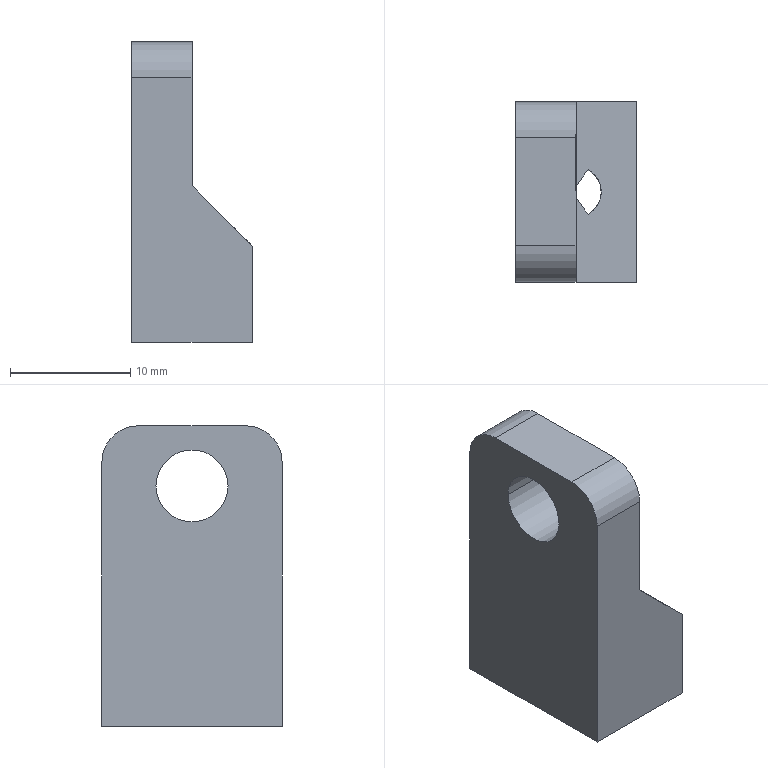Component | SolidWorks | UpperHinge-1 | 1 solid | 15 faces | box 10 x 15 x 25 mm | volume 2332 mm3 | plane 8 | cylinder 6 | cone 1 | commonest cylinder face diameters 6 x4 4.2 x2
STEP:
#1=COLOUR_RGB('',0.7922,0.8196,0.9333);
#2=FILL_AREA_STYLE_COLOUR('',#1);
#3=FILL_AREA_STYLE('',(#2));
#4=SURFACE_STYLE_FILL_AREA(#3);
#5=SURFACE_SIDE_STYLE('',(#4));
#6=SURFACE_STYLE_USAGE(.BOTH.,#5);
#7=PRESENTATION_STYLE_ASSIGNMENT((#6));
#8=CARTESIAN_POINT('',(-0.1614,-8.631,3.169));
#9=VERTEX_POINT('',#8);
#10=CARTESIAN_POINT('',(-0.03937,-8.558,3.169));
#11=VERTEX_POINT('',#10);
#12=CARTESIAN_POINT('',(-0.07874,-8.631,3.169));
#13=DIRECTION('',(0.,0.,-1.));
#14=DIRECTION('',(1.,0.,0.));
#15=AXIS2_PLACEMENT_3D('',#12,#13,#14);
#16=CIRCLE('',#15,0.08268);
#17=EDGE_CURVE('',#9,#11,#16,.T.);
#18=ORIENTED_EDGE('',*,*,#17,.F.);
#19=CARTESIAN_POINT('',(-0.1614,-8.631,2.697));
#20=VERTEX_POINT('',#19);
#21=CARTESIAN_POINT('',(-0.1614,-8.631,2.697));
#22=DIRECTION('',(0.,0.,-1.));
#23=VECTOR('',#22,39.37);
#24=LINE('',#21,#23);
#25=EDGE_CURVE('',#9,#20,#24,.T.);
#26=ORIENTED_EDGE('',*,*,#25,.T.);
#27=CARTESIAN_POINT('',(0.003937,-8.631,2.697));
#28=VERTEX_POINT('',#27);
#29=CARTESIAN_POINT('',(-0.07874,-8.631,2.697));
#30=DIRECTION('',(0.,0.,-1.));
#31=DIRECTION('',(1.,0.,0.));
#32=AXIS2_PLACEMENT_3D('',#29,#30,#31);
#33=CIRCLE('',#32,0.08268);
#34=EDGE_CURVE('',#20,#28,#33,.T.);
#35=ORIENTED_EDGE('',*,*,#34,.T.);
#36=CARTESIAN_POINT('',(0.003937,-8.631,3.126));
#37=VERTEX_POINT('',#36);
#38=CARTESIAN_POINT('',(0.003937,-8.631,2.697));
#39=DIRECTION('',(0.,0.,-1.));
#40=VECTOR('',#39,39.37);
#41=LINE('',#38,#40);
#42=EDGE_CURVE('',#37,#28,#41,.T.);
#43=ORIENTED_EDGE('',*,*,#42,.F.);
#44=CARTESIAN_POINT('',(0.003937,-8.631,3.126));
#45=CARTESIAN_POINT('',(0.003937,-8.6,3.126));
#46=CARTESIAN_POINT('',(-0.01199,-8.573,3.142));
#47=CARTESIAN_POINT('',(-0.03937,-8.558,3.169));
#48=(BOUNDED_CURVE()B_SPLINE_CURVE(3,(#44,#45,#46,#47),.UNSPECIFIED.,.F.,.F.)B_SPLINE_CURVE_WITH_KNOTS((4,4),(0.,1.074),.UNSPECIFIED.)CURVE()GEOMETRIC_REPRESENTATION_ITEM()RATIONAL_B_SPLINE_CURVE((1.,0.9061,0.9061,1.))REPRESENTATION_ITEM(''));
#49=EDGE_CURVE('',#37,#11,#48,.T.);
#50=ORIENTED_EDGE('',*,*,#49,.T.);
#51=EDGE_LOOP('',(#18,#26,#35,#43,#50));
#52=FACE_OUTER_BOUND('',#51,.T.);
#53=CARTESIAN_POINT('',(-0.07874,-8.631,2.697));
#54=DIRECTION('',(0.,0.,-1.));
#55=DIRECTION('',(1.,0.,0.));
#56=AXIS2_PLACEMENT_3D('',#53,#54,#55);
#57=CYLINDRICAL_SURFACE('',#56,0.08268);
#58=ADVANCED_FACE('',(#52),#57,.F.);
#59=CARTESIAN_POINT('',(-0.2756,-8.513,3.484));
#60=VERTEX_POINT('',#59);
#61=CARTESIAN_POINT('',(-0.2756,-8.749,3.484));
#62=VERTEX_POINT('',#61);
#63=CARTESIAN_POINT('',(-0.2756,-8.631,3.484));
#64=DIRECTION('',(1.,0.,0.));
#65=DIRECTION('',(0.,-1.,0.));
#66=AXIS2_PLACEMENT_3D('',#63,#64,#65);
#67=CIRCLE('',#66,0.1181);
#68=EDGE_CURVE('',#60,#62,#67,.T.);
#69=ORIENTED_EDGE('',*,*,#68,.F.);
#70=CARTESIAN_POINT('',(-0.07874,-8.513,3.484));
#71=VERTEX_POINT('',#70);
#72=CARTESIAN_POINT('',(-0.2756,-8.513,3.484));
#73=DIRECTION('',(1.,0.,0.));
#74=VECTOR('',#73,39.37);
#75=LINE('',#72,#74);
#76=EDGE_CURVE('',#60,#71,#75,.T.);
#77=ORIENTED_EDGE('',*,*,#76,.T.);
#78=CARTESIAN_POINT('',(-0.07874,-8.749,3.484));
#79=VERTEX_POINT('',#78);
#80=CARTESIAN_POINT('',(-0.07874,-8.631,3.484));
#81=DIRECTION('',(1.,0.,0.));
#82=DIRECTION('',(-0.,1.,0.));
#83=AXIS2_PLACEMENT_3D('',#80,#81,#82);
#84=CIRCLE('',#83,0.1181);
#85=EDGE_CURVE('',#71,#79,#84,.T.);
#86=ORIENTED_EDGE('',*,*,#85,.T.);
#87=CARTESIAN_POINT('',(-0.2756,-8.749,3.484));
#88=DIRECTION('',(1.,0.,0.));
#89=VECTOR('',#88,39.37);
#90=LINE('',#87,#89);
#91=EDGE_CURVE('',#62,#79,#90,.T.);
#92=ORIENTED_EDGE('',*,*,#91,.F.);
#93=EDGE_LOOP('',(#69,#77,#86,#92));
#94=FACE_OUTER_BOUND('',#93,.T.);
#95=CARTESIAN_POINT('',(-0.2756,-8.631,3.484));
#96=DIRECTION('',(1.,0.,0.));
#97=DIRECTION('',(0.,-1.,0.));
#98=AXIS2_PLACEMENT_3D('',#95,#96,#97);
#99=CYLINDRICAL_SURFACE('',#98,0.1181);
#100=ADVANCED_FACE('',(#94),#99,.F.);
#101=CARTESIAN_POINT('',(-0.2756,-8.336,2.697));
#102=VERTEX_POINT('',#101);
#103=CARTESIAN_POINT('',(-0.2756,-8.336,3.563));
#104=VERTEX_POINT('',#103);
#105=CARTESIAN_POINT('',(-0.2756,-8.336,3.681));
#106=DIRECTION('',(-0.,-0.,1.));
#107=VECTOR('',#106,39.37);
#108=LINE('',#105,#107);
#109=EDGE_CURVE('',#102,#104,#108,.T.);
#110=ORIENTED_EDGE('',*,*,#109,.T.);
#111=CARTESIAN_POINT('',(-0.07874,-8.336,3.563));
#112=VERTEX_POINT('',#111);
#113=CARTESIAN_POINT('',(0.1181,-8.336,3.563));
#114=DIRECTION('',(1.,0.,0.));
#115=VECTOR('',#114,39.37);
#116=LINE('',#113,#115);
#117=EDGE_CURVE('',#104,#112,#116,.T.);
#118=ORIENTED_EDGE('',*,*,#117,.T.);
#119=CARTESIAN_POINT('',(-0.07874,-8.336,3.209));
#120=VERTEX_POINT('',#119);
#121=CARTESIAN_POINT('',(-0.07874,-8.336,3.681));
#122=DIRECTION('',(0.,0.,-1.));
#123=VECTOR('',#122,39.37);
#124=LINE('',#121,#123);
#125=EDGE_CURVE('',#112,#120,#124,.T.);
#126=ORIENTED_EDGE('',*,*,#125,.T.);
#127=CARTESIAN_POINT('',(0.1181,-8.336,3.012));
#128=VERTEX_POINT('',#127);
#129=CARTESIAN_POINT('',(0.1181,-8.336,3.012));
#130=DIRECTION('',(0.7071,0.,-0.7071));
#131=VECTOR('',#130,39.37);
#132=LINE('',#129,#131);
#133=EDGE_CURVE('',#120,#128,#132,.T.);
#134=ORIENTED_EDGE('',*,*,#133,.T.);
#135=CARTESIAN_POINT('',(0.1181,-8.336,2.697));
#136=VERTEX_POINT('',#135);
#137=CARTESIAN_POINT('',(0.1181,-8.336,3.681));
#138=DIRECTION('',(-0.,-0.,1.));
#139=VECTOR('',#138,39.37);
#140=LINE('',#137,#139);
#141=EDGE_CURVE('',#136,#128,#140,.T.);
#142=ORIENTED_EDGE('',*,*,#141,.F.);
#143=CARTESIAN_POINT('',(0.1181,-8.336,2.697));
#144=DIRECTION('',(-1.,-0.,-0.));
#145=VECTOR('',#144,39.37);
#146=LINE('',#143,#145);
#147=EDGE_CURVE('',#136,#102,#146,.T.);
#148=ORIENTED_EDGE('',*,*,#147,.T.);
#149=EDGE_LOOP('',(#110,#118,#126,#134,#142,#148));
#150=FACE_OUTER_BOUND('',#149,.T.);
#151=CARTESIAN_POINT('',(0.1181,-8.336,3.681));
#152=DIRECTION('',(0.,-1.,-0.));
#153=DIRECTION('',(0.,0.,-1.));
#154=AXIS2_PLACEMENT_3D('',#151,#152,#153);
#155=PLANE('',#154);
#156=ADVANCED_FACE('',(#150),#155,.F.);
#157=CARTESIAN_POINT('',(-0.07874,-8.454,3.681));
#158=VERTEX_POINT('',#157);
#159=CARTESIAN_POINT('',(-0.07874,-8.808,3.681));
#160=VERTEX_POINT('',#159);
#161=CARTESIAN_POINT('',(-0.07874,-8.336,3.681));
#162=DIRECTION('',(0.,-1.,-0.));
#163=VECTOR('',#162,39.37);
#164=LINE('',#161,#163);
#165=EDGE_CURVE('',#158,#160,#164,.T.);
#166=ORIENTED_EDGE('',*,*,#165,.F.);
#167=CARTESIAN_POINT('',(-0.2756,-8.454,3.681));
#168=VERTEX_POINT('',#167);
#169=CARTESIAN_POINT('',(0.1181,-8.454,3.681));
#170=DIRECTION('',(-1.,-0.,-0.));
#171=VECTOR('',#170,39.37);
#172=LINE('',#169,#171);
#173=EDGE_CURVE('',#158,#168,#172,.T.);
#174=ORIENTED_EDGE('',*,*,#173,.T.);
#175=CARTESIAN_POINT('',(-0.2756,-8.808,3.681));
#176=VERTEX_POINT('',#175);
#177=CARTESIAN_POINT('',(-0.2756,-8.336,3.681));
#178=DIRECTION('',(0.,-1.,-0.));
#179=VECTOR('',#178,39.37);
#180=LINE('',#177,#179);
#181=EDGE_CURVE('',#168,#176,#180,.T.);
#182=ORIENTED_EDGE('',*,*,#181,.T.);
#183=CARTESIAN_POINT('',(0.1181,-8.808,3.681));
#184=DIRECTION('',(1.,0.,0.));
#185=VECTOR('',#184,39.37);
#186=LINE('',#183,#185);
#187=EDGE_CURVE('',#176,#160,#186,.T.);
#188=ORIENTED_EDGE('',*,*,#187,.T.);
#189=EDGE_LOOP('',(#166,#174,#182,#188));
#190=FACE_OUTER_BOUND('',#189,.T.);
#191=CARTESIAN_POINT('',(0.1181,-8.336,3.681));
#192=DIRECTION('',(0.,0.,-1.));
#193=DIRECTION('',(1.,0.,0.));
#194=AXIS2_PLACEMENT_3D('',#191,#192,#193);
#195=PLANE('',#194);
#196=ADVANCED_FACE('',(#190),#195,.F.);
#197=CARTESIAN_POINT('',(-0.07874,-8.926,3.563));
#198=VERTEX_POINT('',#197);
#199=CARTESIAN_POINT('',(-0.07874,-8.926,3.209));
#200=VERTEX_POINT('',#199);
#201=CARTESIAN_POINT('',(-0.07874,-8.926,3.681));
#202=DIRECTION('',(0.,0.,-1.));
#203=VECTOR('',#202,39.37);
#204=LINE('',#201,#203);
#205=EDGE_CURVE('',#198,#200,#204,.T.);
#206=ORIENTED_EDGE('',*,*,#205,.F.);
#207=CARTESIAN_POINT('',(-0.2756,-8.926,3.563));
#208=VERTEX_POINT('',#207);
#209=CARTESIAN_POINT('',(0.1181,-8.926,3.563));
#210=DIRECTION('',(-1.,-0.,-0.));
#211=VECTOR('',#210,39.37);
#212=LINE('',#209,#211);
#213=EDGE_CURVE('',#198,#208,#212,.T.);
#214=ORIENTED_EDGE('',*,*,#213,.T.);
#215=CARTESIAN_POINT('',(-0.2756,-8.926,2.697));
#216=VERTEX_POINT('',#215);
#217=CARTESIAN_POINT('',(-0.2756,-8.926,3.681));
#218=DIRECTION('',(0.,0.,-1.));
#219=VECTOR('',#218,39.37);
#220=LINE('',#217,#219);
#221=EDGE_CURVE('',#208,#216,#220,.T.);
#222=ORIENTED_EDGE('',*,*,#221,.T.);
#223=CARTESIAN_POINT('',(0.1181,-8.926,2.697));
#224=VERTEX_POINT('',#223);
#225=CARTESIAN_POINT('',(0.1181,-8.926,2.697));
#226=DIRECTION('',(-1.,-0.,-0.));
#227=VECTOR('',#226,39.37);
#228=LINE('',#225,#227);
#229=EDGE_CURVE('',#224,#216,#228,.T.);
#230=ORIENTED_EDGE('',*,*,#229,.F.);
#231=CARTESIAN_POINT('',(0.1181,-8.926,3.012));
#232=VERTEX_POINT('',#231);
#233=CARTESIAN_POINT('',(0.1181,-8.926,3.681));
#234=DIRECTION('',(0.,0.,-1.));
#235=VECTOR('',#234,39.37);
#236=LINE('',#233,#235);
#237=EDGE_CURVE('',#232,#224,#236,.T.);
#238=ORIENTED_EDGE('',*,*,#237,.F.);
#239=CARTESIAN_POINT('',(0.1181,-8.926,3.012));
#240=DIRECTION('',(-0.7071,-0.,0.7071));
#241=VECTOR('',#240,39.37);
#242=LINE('',#239,#241);
#243=EDGE_CURVE('',#232,#200,#242,.T.);
#244=ORIENTED_EDGE('',*,*,#243,.T.);
#245=EDGE_LOOP('',(#206,#214,#222,#230,#238,#244));
#246=FACE_OUTER_BOUND('',#245,.T.);
#247=CARTESIAN_POINT('',(0.1181,-8.926,3.681));
#248=DIRECTION('',(-0.,1.,0.));
#249=DIRECTION('',(-0.,-0.,1.));
#250=AXIS2_PLACEMENT_3D('',#247,#248,#249);
#251=PLANE('',#250);
#252=ADVANCED_FACE('',(#246),#251,.F.);
#253=CARTESIAN_POINT('',(-0.07874,-8.631,2.697));
#254=DIRECTION('',(0.,0.,-1.));
#255=DIRECTION('',(1.,0.,0.));
#256=AXIS2_PLACEMENT_3D('',#253,#254,#255);
#257=CIRCLE('',#256,0.08268);
#258=EDGE_CURVE('',#28,#20,#257,.T.);
#259=ORIENTED_EDGE('',*,*,#258,.F.);
#260=ORIENTED_EDGE('',*,*,#34,.F.);
#261=EDGE_LOOP('',(#259,#260));
#262=FACE_BOUND('',#261,.T.);
#263=CARTESIAN_POINT('',(-0.2756,-8.336,2.697));
#264=DIRECTION('',(-0.,1.,0.));
#265=VECTOR('',#264,39.37);
#266=LINE('',#263,#265);
#267=EDGE_CURVE('',#216,#102,#266,.T.);
#268=ORIENTED_EDGE('',*,*,#267,.T.);
#269=ORIENTED_EDGE('',*,*,#147,.F.);
#270=CARTESIAN_POINT('',(0.1181,-8.336,2.697));
#271=DIRECTION('',(-0.,1.,0.));
#272=VECTOR('',#271,39.37);
#273=LINE('',#270,#272);
#274=EDGE_CURVE('',#224,#136,#273,.T.);
#275=ORIENTED_EDGE('',*,*,#274,.F.);
#276=ORIENTED_EDGE('',*,*,#229,.T.);
#277=EDGE_LOOP('',(#268,#269,#275,#276));
#278=FACE_OUTER_BOUND('',#277,.T.);
#279=CARTESIAN_POINT('',(0.1181,-8.336,2.697));
#280=DIRECTION('',(-0.,-0.,1.));
#281=DIRECTION('',(-1.,-0.,-0.));
#282=AXIS2_PLACEMENT_3D('',#279,#280,#281);
#283=PLANE('',#282);
#284=ADVANCED_FACE('',(#262,#278),#283,.F.);
#285=ORIENTED_EDGE('',*,*,#141,.T.);
#286=CARTESIAN_POINT('',(0.1181,-8.336,3.012));
#287=DIRECTION('',(0.,-1.,-0.));
#288=VECTOR('',#287,39.37);
#289=LINE('',#286,#288);
#290=EDGE_CURVE('',#128,#232,#289,.T.);
#291=ORIENTED_EDGE('',*,*,#290,.T.);
#292=ORIENTED_EDGE('',*,*,#237,.T.);
#293=ORIENTED_EDGE('',*,*,#274,.T.);
#294=EDGE_LOOP('',(#285,#291,#292,#293));
#295=FACE_OUTER_BOUND('',#294,.T.);
#296=CARTESIAN_POINT('',(0.1181,-8.336,3.681));
#297=DIRECTION('',(-1.,-0.,-0.));
#298=DIRECTION('',(-0.,1.,0.));
#299=AXIS2_PLACEMENT_3D('',#296,#297,#298);
#300=PLANE('',#299);
#301=ADVANCED_FACE('',(#295),#300,.F.);
#302=CARTESIAN_POINT('',(-0.2756,-8.631,3.484));
#303=DIRECTION('',(1.,0.,0.));
#304=DIRECTION('',(0.,-1.,0.));
#305=AXIS2_PLACEMENT_3D('',#302,#303,#304);
#306=CIRCLE('',#305,0.1181);
#307=EDGE_CURVE('',#62,#60,#306,.T.);
#308=ORIENTED_EDGE('',*,*,#307,.T.);
#309=ORIENTED_EDGE('',*,*,#68,.T.);
#310=EDGE_LOOP('',(#308,#309));
#311=FACE_BOUND('',#310,.T.);
#312=ORIENTED_EDGE('',*,*,#181,.F.);
#313=CARTESIAN_POINT('',(-0.2756,-8.454,3.563));
#314=DIRECTION('',(-1.,-0.,-0.));
#315=DIRECTION('',(0.,1.,0.));
#316=AXIS2_PLACEMENT_3D('',#313,#314,#315);
#317=CIRCLE('',#316,0.1181);
#318=EDGE_CURVE('',#168,#104,#317,.T.);
#319=ORIENTED_EDGE('',*,*,#318,.T.);
#320=ORIENTED_EDGE('',*,*,#109,.F.);
#321=ORIENTED_EDGE('',*,*,#267,.F.);
#322=ORIENTED_EDGE('',*,*,#221,.F.);
#323=CARTESIAN_POINT('',(-0.2756,-8.808,3.563));
#324=DIRECTION('',(-1.,-0.,-0.));
#325=DIRECTION('',(0.,1.,0.));
#326=AXIS2_PLACEMENT_3D('',#323,#324,#325);
#327=CIRCLE('',#326,0.1181);
#328=EDGE_CURVE('',#208,#176,#327,.T.);
#329=ORIENTED_EDGE('',*,*,#328,.T.);
#330=EDGE_LOOP('',(#312,#319,#320,#321,#322,#329));
#331=FACE_OUTER_BOUND('',#330,.T.);
#332=CARTESIAN_POINT('',(-0.2756,-8.336,3.681));
#333=DIRECTION('',(-1.,-0.,-0.));
#334=DIRECTION('',(-0.,1.,0.));
#335=AXIS2_PLACEMENT_3D('',#332,#333,#334);
#336=PLANE('',#335);
#337=ADVANCED_FACE('',(#311,#331),#336,.T.);
#338=ORIENTED_EDGE('',*,*,#76,.F.);
#339=ORIENTED_EDGE('',*,*,#307,.F.);
#340=ORIENTED_EDGE('',*,*,#91,.T.);
#341=CARTESIAN_POINT('',(-0.07874,-8.631,3.484));
#342=DIRECTION('',(1.,0.,0.));
#343=DIRECTION('',(-0.,1.,0.));
#344=AXIS2_PLACEMENT_3D('',#341,#342,#343);
#345=CIRCLE('',#344,0.1181);
#346=EDGE_CURVE('',#79,#71,#345,.T.);
#347=ORIENTED_EDGE('',*,*,#346,.T.);
#348=EDGE_LOOP('',(#338,#339,#340,#347));
#349=FACE_OUTER_BOUND('',#348,.T.);
#350=CARTESIAN_POINT('',(-0.2756,-8.631,3.484));
#351=DIRECTION('',(1.,0.,0.));
#352=DIRECTION('',(0.,-1.,0.));
#353=AXIS2_PLACEMENT_3D('',#350,#351,#352);
#354=CYLINDRICAL_SURFACE('',#353,0.1181);
#355=ADVANCED_FACE('',(#349),#354,.F.);
#356=ORIENTED_EDGE('',*,*,#125,.F.);
#357=CARTESIAN_POINT('',(-0.07874,-8.454,3.563));
#358=DIRECTION('',(1.,0.,0.));
#359=DIRECTION('',(-0.,1.,0.));
#360=AXIS2_PLACEMENT_3D('',#357,#358,#359);
#361=CIRCLE('',#360,0.1181);
#362=EDGE_CURVE('',#112,#158,#361,.T.);
#363=ORIENTED_EDGE('',*,*,#362,.T.);
#364=ORIENTED_EDGE('',*,*,#165,.T.);
#365=CARTESIAN_POINT('',(-0.07874,-8.808,3.563));
#366=DIRECTION('',(1.,0.,0.));
#367=DIRECTION('',(-0.,1.,0.));
#368=AXIS2_PLACEMENT_3D('',#365,#366,#367);
#369=CIRCLE('',#368,0.1181);
#370=EDGE_CURVE('',#160,#198,#369,.T.);
#371=ORIENTED_EDGE('',*,*,#370,.T.);
#372=ORIENTED_EDGE('',*,*,#205,.T.);
#373=CARTESIAN_POINT('',(-0.07874,-8.648,3.209));
#374=VERTEX_POINT('',#373);
#375=CARTESIAN_POINT('',(-0.07874,-8.336,3.209));
#376=DIRECTION('',(0.,-1.,-0.));
#377=VECTOR('',#376,39.37);
#378=LINE('',#375,#377);
#379=EDGE_CURVE('',#374,#200,#378,.T.);
#380=ORIENTED_EDGE('',*,*,#379,.F.);
#381=CARTESIAN_POINT('',(-0.07874,-8.631,3.219));
#382=VERTEX_POINT('',#381);
#383=CARTESIAN_POINT('',(-0.07874,-8.631,3.219));
#384=DIRECTION('',(-0.,0.8572,0.515));
#385=VECTOR('',#384,39.37);
#386=LINE('',#383,#385);
#387=EDGE_CURVE('',#374,#382,#386,.T.);
#388=ORIENTED_EDGE('',*,*,#387,.T.);
#389=CARTESIAN_POINT('',(-0.07874,-8.614,3.209));
#390=VERTEX_POINT('',#389);
#391=CARTESIAN_POINT('',(-0.07874,-8.631,3.219));
#392=DIRECTION('',(-0.,0.8572,-0.515));
#393=VECTOR('',#392,39.37);
#394=LINE('',#391,#393);
#395=EDGE_CURVE('',#382,#390,#394,.T.);
#396=ORIENTED_EDGE('',*,*,#395,.T.);
#397=CARTESIAN_POINT('',(-0.07874,-8.336,3.209));
#398=DIRECTION('',(0.,-1.,-0.));
#399=VECTOR('',#398,39.37);
#400=LINE('',#397,#399);
#401=EDGE_CURVE('',#120,#390,#400,.T.);
#402=ORIENTED_EDGE('',*,*,#401,.F.);
#403=EDGE_LOOP('',(#356,#363,#364,#371,#372,#380,#388,#396,#402));
#404=FACE_OUTER_BOUND('',#403,.T.);
#405=ORIENTED_EDGE('',*,*,#346,.F.);
#406=ORIENTED_EDGE('',*,*,#85,.F.);
#407=EDGE_LOOP('',(#405,#406));
#408=FACE_BOUND('',#407,.T.);
#409=CARTESIAN_POINT('',(-0.07874,-8.336,3.681));
#410=DIRECTION('',(-1.,-0.,-0.));
#411=DIRECTION('',(-0.,1.,0.));
#412=AXIS2_PLACEMENT_3D('',#409,#410,#411);
#413=PLANE('',#412);
#414=ADVANCED_FACE('',(#404,#408),#413,.F.);
#415=ORIENTED_EDGE('',*,*,#387,.F.);
#416=CARTESIAN_POINT('',(-0.03937,-8.704,3.169));
#417=VERTEX_POINT('',#416);
#418=CARTESIAN_POINT('',(-0.07874,-8.648,3.209));
#419=CARTESIAN_POINT('',(-0.07574,-8.653,3.206));
#420=CARTESIAN_POINT('',(-0.07251,-8.658,3.202));
#421=CARTESIAN_POINT('',(-0.06601,-8.667,3.196));
#422=CARTESIAN_POINT('',(-0.06271,-8.672,3.193));
#423=CARTESIAN_POINT('',(-0.05277,-8.686,3.183));
#424=CARTESIAN_POINT('',(-0.04607,-8.695,3.176));
#425=CARTESIAN_POINT('',(-0.03937,-8.704,3.169));
#426=B_SPLINE_CURVE_WITH_KNOTS('',3,(#418,#419,#420,#421,#422,#423,#424,#425),.UNSPECIFIED.,.F.,.F.,(4,2,2,4),(0.,0.0004995,0.000999,0.001998),.UNSPECIFIED.);
#427=EDGE_CURVE('',#374,#417,#426,.T.);
#428=ORIENTED_EDGE('',*,*,#427,.T.);
#429=CARTESIAN_POINT('',(-0.07874,-8.631,3.169));
#430=DIRECTION('',(0.,0.,-1.));
#431=DIRECTION('',(1.,0.,0.));
#432=AXIS2_PLACEMENT_3D('',#429,#430,#431);
#433=CIRCLE('',#432,0.08268);
#434=EDGE_CURVE('',#417,#9,#433,.T.);
#435=ORIENTED_EDGE('',*,*,#434,.T.);
#436=ORIENTED_EDGE('',*,*,#17,.T.);
#437=CARTESIAN_POINT('',(-0.03937,-8.558,3.169));
#438=CARTESIAN_POINT('',(-0.04607,-8.567,3.176));
#439=CARTESIAN_POINT('',(-0.05277,-8.576,3.183));
#440=CARTESIAN_POINT('',(-0.06271,-8.59,3.193));
#441=CARTESIAN_POINT('',(-0.06601,-8.595,3.196));
#442=CARTESIAN_POINT('',(-0.07251,-8.604,3.202));
#443=CARTESIAN_POINT('',(-0.07574,-8.609,3.206));
#444=CARTESIAN_POINT('',(-0.07874,-8.614,3.209));
#445=B_SPLINE_CURVE_WITH_KNOTS('',3,(#437,#438,#439,#440,#441,#442,#443,#444),.UNSPECIFIED.,.F.,.F.,(4,2,2,4),(0.,0.0009991,0.001499,0.001998),.UNSPECIFIED.);
#446=EDGE_CURVE('',#11,#390,#445,.T.);
#447=ORIENTED_EDGE('',*,*,#446,.T.);
#448=ORIENTED_EDGE('',*,*,#395,.F.);
#449=EDGE_LOOP('',(#415,#428,#435,#436,#447,#448));
#450=FACE_OUTER_BOUND('',#449,.T.);
#451=CARTESIAN_POINT('',(-0.07874,-8.631,3.169));
#452=DIRECTION('',(0.,0.,-1.));
#453=DIRECTION('',(1.,0.,0.));
#454=AXIS2_PLACEMENT_3D('',#451,#452,#453);
#455=CONICAL_SURFACE('',#454,0.08268,1.03);
#456=ADVANCED_FACE('',(#450),#455,.F.);
#457=ORIENTED_EDGE('',*,*,#25,.F.);
#458=ORIENTED_EDGE('',*,*,#434,.F.);
#459=CARTESIAN_POINT('',(-0.03937,-8.704,3.169));
#460=CARTESIAN_POINT('',(-0.01199,-8.689,3.142));
#461=CARTESIAN_POINT('',(0.003937,-8.662,3.126));
#462=CARTESIAN_POINT('',(0.003937,-8.631,3.126));
#463=(BOUNDED_CURVE()B_SPLINE_CURVE(3,(#459,#460,#461,#462),.UNSPECIFIED.,.F.,.F.)B_SPLINE_CURVE_WITH_KNOTS((4,4),(5.209,6.283),.UNSPECIFIED.)CURVE()GEOMETRIC_REPRESENTATION_ITEM()RATIONAL_B_SPLINE_CURVE((1.,0.9061,0.9061,1.))REPRESENTATION_ITEM(''));
#464=EDGE_CURVE('',#417,#37,#463,.T.);
#465=ORIENTED_EDGE('',*,*,#464,.T.);
#466=ORIENTED_EDGE('',*,*,#42,.T.);
#467=ORIENTED_EDGE('',*,*,#258,.T.);
#468=EDGE_LOOP('',(#457,#458,#465,#466,#467));
#469=FACE_OUTER_BOUND('',#468,.T.);
#470=CARTESIAN_POINT('',(-0.07874,-8.631,2.697));
#471=DIRECTION('',(0.,0.,-1.));
#472=DIRECTION('',(1.,0.,0.));
#473=AXIS2_PLACEMENT_3D('',#470,#471,#472);
#474=CYLINDRICAL_SURFACE('',#473,0.08268);
#475=ADVANCED_FACE('',(#469),#474,.F.);
#476=ORIENTED_EDGE('',*,*,#427,.F.);
#477=ORIENTED_EDGE('',*,*,#379,.T.);
#478=ORIENTED_EDGE('',*,*,#243,.F.);
#479=ORIENTED_EDGE('',*,*,#290,.F.);
#480=ORIENTED_EDGE('',*,*,#133,.F.);
#481=ORIENTED_EDGE('',*,*,#401,.T.);
#482=ORIENTED_EDGE('',*,*,#446,.F.);
#483=ORIENTED_EDGE('',*,*,#49,.F.);
#484=ORIENTED_EDGE('',*,*,#464,.F.);
#485=EDGE_LOOP('',(#476,#477,#478,#479,#480,#481,#482,#483,#484));
#486=FACE_OUTER_BOUND('',#485,.T.);
#487=CARTESIAN_POINT('',(0.1181,-8.336,3.012));
#488=DIRECTION('',(-0.7071,0.,-0.7071));
#489=DIRECTION('',(0.,-1.,-0.));
#490=AXIS2_PLACEMENT_3D('',#487,#488,#489);
#491=PLANE('',#490);
#492=ADVANCED_FACE('',(#486),#491,.F.);
#493=ORIENTED_EDGE('',*,*,#362,.F.);
#494=ORIENTED_EDGE('',*,*,#117,.F.);
#495=ORIENTED_EDGE('',*,*,#318,.F.);
#496=ORIENTED_EDGE('',*,*,#173,.F.);
#497=EDGE_LOOP('',(#493,#494,#495,#496));
#498=FACE_OUTER_BOUND('',#497,.T.);
#499=CARTESIAN_POINT('',(0.1181,-8.454,3.563));
#500=DIRECTION('',(-1.,-0.,-0.));
#501=DIRECTION('',(-0.,1.,0.));
#502=AXIS2_PLACEMENT_3D('',#499,#500,#501);
#503=CYLINDRICAL_SURFACE('',#502,0.1181);
#504=ADVANCED_FACE('',(#498),#503,.T.);
#505=ORIENTED_EDGE('',*,*,#370,.F.);
#506=ORIENTED_EDGE('',*,*,#187,.F.);
#507=ORIENTED_EDGE('',*,*,#328,.F.);
#508=ORIENTED_EDGE('',*,*,#213,.F.);
#509=EDGE_LOOP('',(#505,#506,#507,#508));
#510=FACE_OUTER_BOUND('',#509,.T.);
#511=CARTESIAN_POINT('',(0.1181,-8.808,3.563));
#512=DIRECTION('',(-1.,-0.,-0.));
#513=DIRECTION('',(-0.,1.,0.));
#514=AXIS2_PLACEMENT_3D('',#511,#512,#513);
#515=CYLINDRICAL_SURFACE('',#514,0.1181);
#516=ADVANCED_FACE('',(#510),#515,.T.);
#517=CLOSED_SHELL('',(#58,#100,#156,#196,#252,#284,#301,#337,#355,#414,#456,#475,#492,#504,#516));
#518=MANIFOLD_SOLID_BREP('',#517);
#519=STYLED_ITEM('',(#7),#518);
#520=PRESENTATION_LAYER_ASSIGNMENT('','',(#519));
#521=CARTESIAN_POINT('',(0.,0.,0.));
#522=DIRECTION('',(0.,0.,1.));
#523=DIRECTION('',(1.,0.,0.));
#524=AXIS2_PLACEMENT_3D('',#521,#522,#523);
#525=(LENGTH_UNIT()NAMED_UNIT(*)SI_UNIT($,.METRE.));
#526=LENGTH_MEASURE_WITH_UNIT(LENGTH_MEASURE(0.0254),#525);
#527=DIMENSIONAL_EXPONENTS(1.,0.,0.,0.,0.,0.,0.);
#528=(CONVERSION_BASED_UNIT('',#526)LENGTH_UNIT()NAMED_UNIT(#527));
#529=UNCERTAINTY_MEASURE_WITH_UNIT(LENGTH_MEASURE(0.00001),#528,'','');
#530=(NAMED_UNIT(*)PLANE_ANGLE_UNIT()SI_UNIT($,.RADIAN.));
#531=(NAMED_UNIT(*)SI_UNIT($,.STERADIAN.)SOLID_ANGLE_UNIT());
#532=(GEOMETRIC_REPRESENTATION_CONTEXT(3)GLOBAL_UNCERTAINTY_ASSIGNED_CONTEXT((#529))GLOBAL_UNIT_ASSIGNED_CONTEXT((#528,#530,#531))REPRESENTATION_CONTEXT('',''));
#533=ADVANCED_BREP_SHAPE_REPRESENTATION('',(#518,#524),#532);
#534=(LENGTH_UNIT()NAMED_UNIT(*)SI_UNIT($,.METRE.));
#535=LENGTH_MEASURE_WITH_UNIT(LENGTH_MEASURE(0.0254),#534);
#536=DIMENSIONAL_EXPONENTS(1.,0.,0.,0.,0.,0.,0.);
#537=(CONVERSION_BASED_UNIT('',#535)LENGTH_UNIT()NAMED_UNIT(#536));
#538=UNCERTAINTY_MEASURE_WITH_UNIT(LENGTH_MEASURE(0.00001),#537,'','');
#539=(NAMED_UNIT(*)PLANE_ANGLE_UNIT()SI_UNIT($,.RADIAN.));
#540=(NAMED_UNIT(*)SI_UNIT($,.STERADIAN.)SOLID_ANGLE_UNIT());
#541=(GEOMETRIC_REPRESENTATION_CONTEXT(3)GLOBAL_UNCERTAINTY_ASSIGNED_CONTEXT((#538))GLOBAL_UNIT_ASSIGNED_CONTEXT((#537,#539,#540))REPRESENTATION_CONTEXT('',''));
#542=MECHANICAL_DESIGN_GEOMETRIC_PRESENTATION_REPRESENTATION('',(#519),#541);